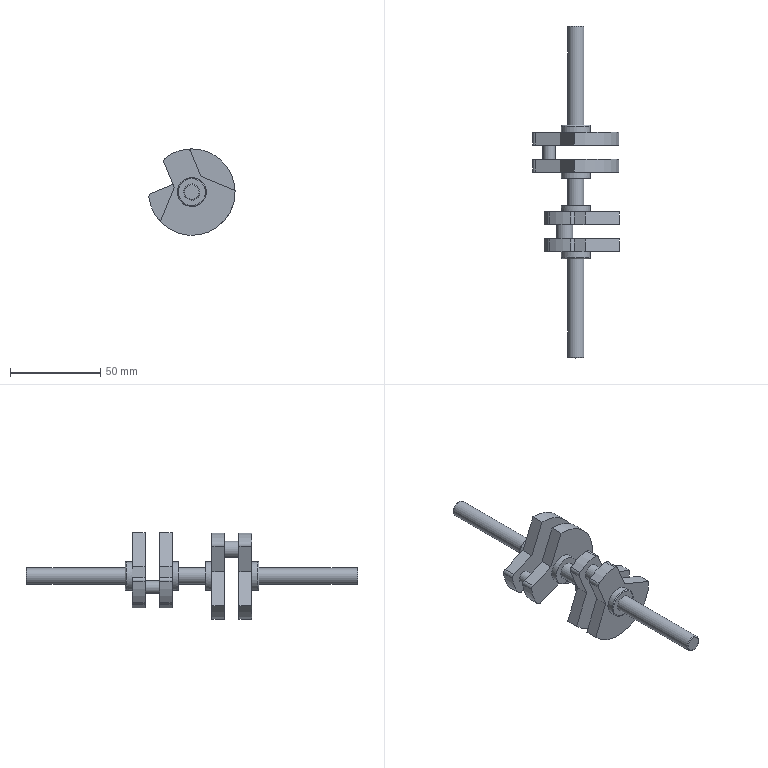Component | NX | CRANKSHAFT | 1 solid | 59 faces | volume 46151 mm3 | plane 30 | cylinder 25 | torus 4 | commonest cylinder face diameters 48 x8 4 x8 9 x4 16 x4 7 x1